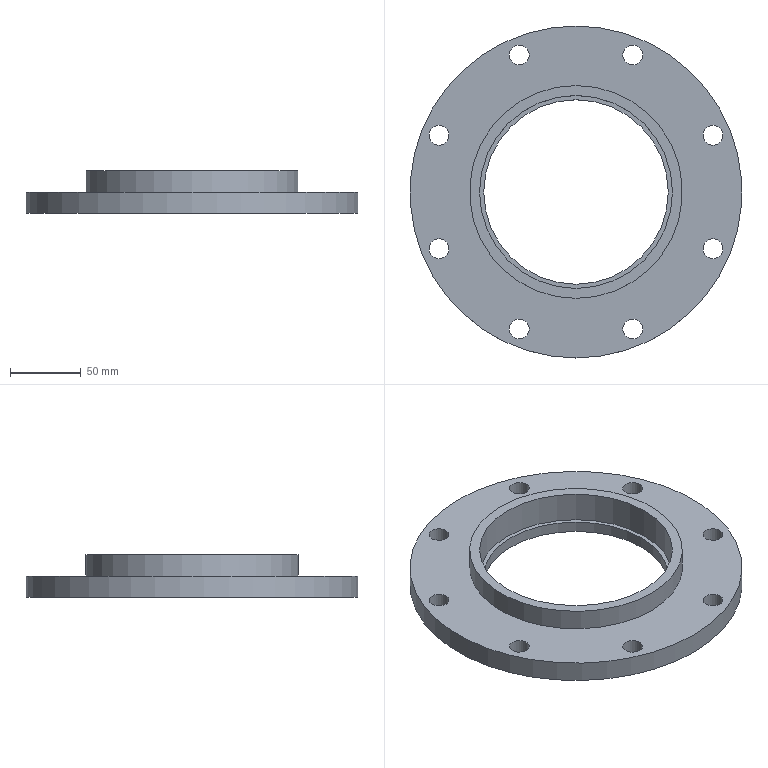Component | NX | CH3404-12 | 1 solid | 16 faces | volume 465904 mm3 | cylinder 12 | plane 4 | commonest cylinder face diameters 14 x8 130 x1 234 x1 150 x1 136 x1